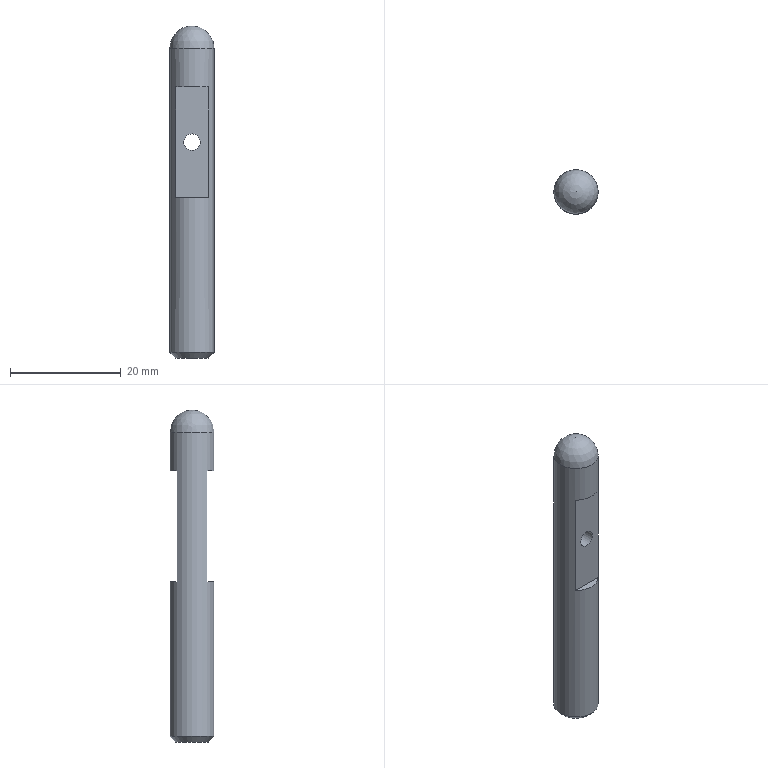Component | NX | ADJ_SUPPORT | 1 solid | 11 faces | box 8 x 8 x 60 mm | volume 2687 mm3 | plane 7 | cylinder 2 | sphere 1 | cone 1 | commonest cylinder face diameters 8 x1 3 x1
STEP:
#1=CARTESIAN_POINT('',(0.,0.,0.));
#2=DIRECTION('',(0.,0.,1.));
#3=DIRECTION('',(1.,0.,0.));
#4=AXIS2_PLACEMENT_3D('',#1,#2,#3);
#5=CARTESIAN_POINT('',(-84.,70.,-253.));
#6=VERTEX_POINT('',#5);
#7=CARTESIAN_POINT('',(-92.,70.,-253.));
#8=VERTEX_POINT('',#7);
#9=CARTESIAN_POINT('',(-88.,70.,-253.));
#10=DIRECTION('',(0.,0.,1.));
#11=DIRECTION('',(1.,0.,0.));
#12=AXIS2_PLACEMENT_3D('',#9,#10,#11);
#13=CIRCLE('',#12,4.);
#14=CARTESIAN_POINT('',(-88.,70.,-254.));
#15=DIRECTION('',(0.,0.,1.));
#16=DIRECTION('',(-1.,0.,0.));
#17=AXIS2_PLACEMENT_3D('',#14,#15,#16);
#18=CYLINDRICAL_SURFACE('',#17,4.);
#19=CARTESIAN_POINT('',(3.142,1.));
#20=DIRECTION('',(1.,0.));
#21=VECTOR('',#20,1.);
#22=LINE('',#19,#21);
#23=(GEOMETRIC_REPRESENTATION_CONTEXT(2)PARAMETRIC_REPRESENTATION_CONTEXT()REPRESENTATION_CONTEXT('',''));
#24=DEFINITIONAL_REPRESENTATION('',(#22),#23);
#25=PCURVE('',#18,#24);
#26=CARTESIAN_POINT('',(-88.,70.,-253.));
#27=DIRECTION('',(0.,0.,1.));
#28=DIRECTION('',(-1.,0.,0.));
#29=AXIS2_PLACEMENT_3D('',#26,#27,#28);
#30=CONICAL_SURFACE('',#29,4.,0.7854);
#31=CARTESIAN_POINT('',(3.142,0.));
#32=DIRECTION('',(1.,0.));
#33=VECTOR('',#32,1.);
#34=LINE('',#31,#33);
#35=(GEOMETRIC_REPRESENTATION_CONTEXT(2)PARAMETRIC_REPRESENTATION_CONTEXT()REPRESENTATION_CONTEXT('',''));
#36=DEFINITIONAL_REPRESENTATION('',(#34),#35);
#37=PCURVE('',#30,#36);
#38=SURFACE_CURVE('',#13,(#25,#37),.PCURVE_S1.);
#39=EDGE_CURVE('',#6,#8,#38,.T.);
#40=ORIENTED_EDGE('',*,*,#39,.T.);
#41=CARTESIAN_POINT('',(-92.,70.,-198.));
#42=VERTEX_POINT('',#41);
#43=CARTESIAN_POINT('',(-92.,70.,-253.));
#44=CARTESIAN_POINT('',(-92.,70.,-198.));
#45=B_SPLINE_CURVE_WITH_KNOTS('',1,(#43,#44),.UNSPECIFIED.,.F.,.F.,(2,2),(1.,56.),.PIECEWISE_BEZIER_KNOTS.);
#46=CARTESIAN_POINT('',(6.283,0.));
#47=DIRECTION('',(0.,1.));
#48=VECTOR('',#47,1.);
#49=LINE('',#46,#48);
#50=(GEOMETRIC_REPRESENTATION_CONTEXT(2)PARAMETRIC_REPRESENTATION_CONTEXT()REPRESENTATION_CONTEXT('',''));
#51=DEFINITIONAL_REPRESENTATION('',(#49),#50);
#52=PCURVE('',#18,#51);
#53=CARTESIAN_POINT('',(0.,0.));
#54=DIRECTION('',(0.,1.));
#55=VECTOR('',#54,1.);
#56=LINE('',#53,#55);
#57=(GEOMETRIC_REPRESENTATION_CONTEXT(2)PARAMETRIC_REPRESENTATION_CONTEXT()REPRESENTATION_CONTEXT('',''));
#58=DEFINITIONAL_REPRESENTATION('',(#56),#57);
#59=PCURVE('',#18,#58);
#60=SEAM_CURVE('',#45,(#52,#59),.PCURVE_S1.);
#61=EDGE_CURVE('',#8,#42,#60,.T.);
#62=ORIENTED_EDGE('',*,*,#61,.T.);
#63=CARTESIAN_POINT('',(-88.,70.,-198.));
#64=DIRECTION('',(0.,0.,-1.));
#65=DIRECTION('',(-1.,0.,0.));
#66=AXIS2_PLACEMENT_3D('',#63,#64,#65);
#67=CIRCLE('',#66,4.);
#68=CARTESIAN_POINT('',(6.283,56.));
#69=DIRECTION('',(-1.,0.));
#70=VECTOR('',#69,1.);
#71=LINE('',#68,#70);
#72=(GEOMETRIC_REPRESENTATION_CONTEXT(2)PARAMETRIC_REPRESENTATION_CONTEXT()REPRESENTATION_CONTEXT('',''));
#73=DEFINITIONAL_REPRESENTATION('',(#71),#72);
#74=PCURVE('',#18,#73);
#75=CARTESIAN_POINT('',(-88.,70.,-198.));
#76=DIRECTION('',(0.,0.,1.));
#77=DIRECTION('',(-1.,0.,0.));
#78=AXIS2_PLACEMENT_3D('',#75,#76,#77);
#79=SPHERICAL_SURFACE('',#78,4.);
#80=CARTESIAN_POINT('',(6.283,0.));
#81=CARTESIAN_POINT('',(6.188,0.));
#82=CARTESIAN_POINT('',(5.998,0.));
#83=CARTESIAN_POINT('',(5.712,0.));
#84=CARTESIAN_POINT('',(5.426,0.));
#85=CARTESIAN_POINT('',(5.141,0.));
#86=CARTESIAN_POINT('',(4.855,0.));
#87=CARTESIAN_POINT('',(4.57,0.));
#88=CARTESIAN_POINT('',(4.284,0.));
#89=CARTESIAN_POINT('',(3.998,0.));
#90=CARTESIAN_POINT('',(3.713,0.));
#91=CARTESIAN_POINT('',(3.427,0.));
#92=CARTESIAN_POINT('',(3.142,0.));
#93=CARTESIAN_POINT('',(2.856,0.));
#94=CARTESIAN_POINT('',(2.57,0.));
#95=CARTESIAN_POINT('',(2.285,0.));
#96=CARTESIAN_POINT('',(1.999,0.));
#97=CARTESIAN_POINT('',(1.714,0.));
#98=CARTESIAN_POINT('',(1.428,0.));
#99=CARTESIAN_POINT('',(1.142,0.));
#100=CARTESIAN_POINT('',(0.8568,0.));
#101=CARTESIAN_POINT('',(0.5712,0.));
#102=CARTESIAN_POINT('',(0.2856,0.));
#103=CARTESIAN_POINT('',(0.0952,0.));
#104=CARTESIAN_POINT('',(0.,0.));
#105=B_SPLINE_CURVE_WITH_KNOTS('',3,(#80,#81,#82,#83,#84,#85,#86,#87,#88,#89,#90,#91,#92,#93,#94,#95,#96,#97,#98,#99,#100,#101,#102,#103,#104),.UNSPECIFIED.,.F.,.F.,(4,1,1,1,1,1,1,1,1,1,1,1,1,1,1,1,1,1,1,1,1,1,4),(0.,0.2856,0.5712,0.8568,1.142,1.428,1.714,1.999,2.285,2.57,2.856,3.142,3.427,3.713,3.998,4.284,4.57,4.855,5.141,5.426,5.712,5.998,6.283),.QUASI_UNIFORM_KNOTS.);
#106=(GEOMETRIC_REPRESENTATION_CONTEXT(2)PARAMETRIC_REPRESENTATION_CONTEXT()REPRESENTATION_CONTEXT('',''));
#107=DEFINITIONAL_REPRESENTATION('',(#105),#106);
#108=PCURVE('',#79,#107);
#109=SURFACE_CURVE('',#67,(#74,#108),.PCURVE_S1.);
#110=EDGE_CURVE('',#42,#42,#109,.T.);
#111=ORIENTED_EDGE('',*,*,#110,.T.);
#112=ORIENTED_EDGE('',*,*,#61,.F.);
#113=CARTESIAN_POINT('',(-88.,70.,-253.));
#114=DIRECTION('',(0.,0.,1.));
#115=DIRECTION('',(1.,0.,0.));
#116=AXIS2_PLACEMENT_3D('',#113,#114,#115);
#117=CIRCLE('',#116,4.);
#118=CARTESIAN_POINT('',(-3.142,1.));
#119=DIRECTION('',(1.,0.));
#120=VECTOR('',#119,1.);
#121=LINE('',#118,#120);
#122=(GEOMETRIC_REPRESENTATION_CONTEXT(2)PARAMETRIC_REPRESENTATION_CONTEXT()REPRESENTATION_CONTEXT('',''));
#123=DEFINITIONAL_REPRESENTATION('',(#121),#122);
#124=PCURVE('',#18,#123);
#125=CARTESIAN_POINT('',(3.142,0.));
#126=DIRECTION('',(1.,0.));
#127=VECTOR('',#126,1.);
#128=LINE('',#125,#127);
#129=(GEOMETRIC_REPRESENTATION_CONTEXT(2)PARAMETRIC_REPRESENTATION_CONTEXT()REPRESENTATION_CONTEXT('',''));
#130=DEFINITIONAL_REPRESENTATION('',(#128),#129);
#131=PCURVE('',#30,#130);
#132=SURFACE_CURVE('',#117,(#124,#131),.PCURVE_S1.);
#133=EDGE_CURVE('',#8,#6,#132,.T.);
#134=ORIENTED_EDGE('',*,*,#133,.T.);
#135=EDGE_LOOP('',(#40,#62,#111,#112,#134));
#136=FACE_BOUND('',#135,.T.);
#137=CARTESIAN_POINT('',(-85.049,67.3,-205.));
#138=VERTEX_POINT('',#137);
#139=CARTESIAN_POINT('',(-85.049,67.3,-225.));
#140=VERTEX_POINT('',#139);
#141=CARTESIAN_POINT('',(-85.049,67.3,-254.));
#142=DIRECTION('',(0.,0.,-1.));
#143=VECTOR('',#142,1.);
#144=LINE('',#141,#143);
#145=CARTESIAN_POINT('',(2.401,0.));
#146=DIRECTION('',(0.,-1.));
#147=VECTOR('',#146,1.);
#148=LINE('',#145,#147);
#149=(GEOMETRIC_REPRESENTATION_CONTEXT(2)PARAMETRIC_REPRESENTATION_CONTEXT()REPRESENTATION_CONTEXT('',''));
#150=DEFINITIONAL_REPRESENTATION('',(#148),#149);
#151=PCURVE('',#18,#150);
#152=CARTESIAN_POINT('',(-108.,67.3,-205.));
#153=DIRECTION('',(0.,-1.,0.));
#154=DIRECTION('',(0.,0.,1.));
#155=AXIS2_PLACEMENT_3D('',#152,#153,#154);
#156=PLANE('',#155);
#157=CARTESIAN_POINT('',(-49.,-22.951));
#158=DIRECTION('',(-1.,0.));
#159=VECTOR('',#158,1.);
#160=LINE('',#157,#159);
#161=(GEOMETRIC_REPRESENTATION_CONTEXT(2)PARAMETRIC_REPRESENTATION_CONTEXT()REPRESENTATION_CONTEXT('',''));
#162=DEFINITIONAL_REPRESENTATION('',(#160),#161);
#163=PCURVE('',#156,#162);
#164=SURFACE_CURVE('',#144,(#151,#163),.PCURVE_S1.);
#165=EDGE_CURVE('',#138,#140,#164,.T.);
#166=ORIENTED_EDGE('',*,*,#165,.T.);
#167=CARTESIAN_POINT('',(-90.951,67.3,-225.));
#168=VERTEX_POINT('',#167);
#169=CARTESIAN_POINT('',(-88.,70.,-225.));
#170=DIRECTION('',(0.,0.,-1.));
#171=DIRECTION('',(-1.,0.,0.));
#172=AXIS2_PLACEMENT_3D('',#169,#170,#171);
#173=CIRCLE('',#172,4.);
#174=CARTESIAN_POINT('',(6.283,29.));
#175=DIRECTION('',(-1.,0.));
#176=VECTOR('',#175,1.);
#177=LINE('',#174,#176);
#178=(GEOMETRIC_REPRESENTATION_CONTEXT(2)PARAMETRIC_REPRESENTATION_CONTEXT()REPRESENTATION_CONTEXT('',''));
#179=DEFINITIONAL_REPRESENTATION('',(#177),#178);
#180=PCURVE('',#18,#179);
#181=CARTESIAN_POINT('',(-108.,67.3,-225.));
#182=DIRECTION('',(0.,0.,1.));
#183=DIRECTION('',(-1.,0.,0.));
#184=AXIS2_PLACEMENT_3D('',#181,#182,#183);
#185=PLANE('',#184);
#186=CARTESIAN_POINT('',(-16.,-2.7));
#187=CARTESIAN_POINT('',(-16.,-9.628));
#188=CARTESIAN_POINT('',(-22.,-6.164));
#189=CARTESIAN_POINT('',(-28.,-2.7));
#190=CARTESIAN_POINT('',(-22.,0.7641));
#191=CARTESIAN_POINT('',(-16.,4.228));
#192=CARTESIAN_POINT('',(-16.,-2.7));
#193=(BOUNDED_CURVE()B_SPLINE_CURVE(2,(#186,#187,#188,#189,#190,#191,#192),.UNSPECIFIED.,.T.,.F.)B_SPLINE_CURVE_WITH_KNOTS((1,2,2,2,2,1),(-2.094,0.,2.094,4.189,6.283,8.378),.UNSPECIFIED.)CURVE()GEOMETRIC_REPRESENTATION_ITEM()RATIONAL_B_SPLINE_CURVE((1.,0.5,1.,0.5,1.,0.5,1.))REPRESENTATION_ITEM(''));
#194=(GEOMETRIC_REPRESENTATION_CONTEXT(2)PARAMETRIC_REPRESENTATION_CONTEXT()REPRESENTATION_CONTEXT('',''));
#195=DEFINITIONAL_REPRESENTATION('',(#193),#194);
#196=PCURVE('',#185,#195);
#197=SURFACE_CURVE('',#173,(#180,#196),.PCURVE_S1.);
#198=EDGE_CURVE('',#140,#168,#197,.T.);
#199=ORIENTED_EDGE('',*,*,#198,.T.);
#200=CARTESIAN_POINT('',(-90.951,67.3,-205.));
#201=VERTEX_POINT('',#200);
#202=CARTESIAN_POINT('',(-90.951,67.3,-254.));
#203=DIRECTION('',(0.,0.,1.));
#204=VECTOR('',#203,1.);
#205=LINE('',#202,#204);
#206=CARTESIAN_POINT('',(0.741,0.));
#207=DIRECTION('',(0.,1.));
#208=VECTOR('',#207,1.);
#209=LINE('',#206,#208);
#210=(GEOMETRIC_REPRESENTATION_CONTEXT(2)PARAMETRIC_REPRESENTATION_CONTEXT()REPRESENTATION_CONTEXT('',''));
#211=DEFINITIONAL_REPRESENTATION('',(#209),#210);
#212=PCURVE('',#18,#211);
#213=CARTESIAN_POINT('',(-49.,-17.049));
#214=DIRECTION('',(1.,0.));
#215=VECTOR('',#214,1.);
#216=LINE('',#213,#215);
#217=(GEOMETRIC_REPRESENTATION_CONTEXT(2)PARAMETRIC_REPRESENTATION_CONTEXT()REPRESENTATION_CONTEXT('',''));
#218=DEFINITIONAL_REPRESENTATION('',(#216),#217);
#219=PCURVE('',#156,#218);
#220=SURFACE_CURVE('',#205,(#212,#219),.PCURVE_S1.);
#221=EDGE_CURVE('',#168,#201,#220,.T.);
#222=ORIENTED_EDGE('',*,*,#221,.T.);
#223=CARTESIAN_POINT('',(-88.,70.,-205.));
#224=DIRECTION('',(0.,0.,1.));
#225=DIRECTION('',(1.,0.,0.));
#226=AXIS2_PLACEMENT_3D('',#223,#224,#225);
#227=CIRCLE('',#226,4.);
#228=CARTESIAN_POINT('',(-3.142,49.));
#229=DIRECTION('',(1.,0.));
#230=VECTOR('',#229,1.);
#231=LINE('',#228,#230);
#232=(GEOMETRIC_REPRESENTATION_CONTEXT(2)PARAMETRIC_REPRESENTATION_CONTEXT()REPRESENTATION_CONTEXT('',''));
#233=DEFINITIONAL_REPRESENTATION('',(#231),#232);
#234=PCURVE('',#18,#233);
#235=CARTESIAN_POINT('',(-108.,60.,-205.));
#236=DIRECTION('',(0.,0.,-1.));
#237=DIRECTION('',(1.,0.,0.));
#238=AXIS2_PLACEMENT_3D('',#235,#236,#237);
#239=PLANE('',#238);
#240=CARTESIAN_POINT('',(24.,-10.));
#241=CARTESIAN_POINT('',(24.,-16.928));
#242=CARTESIAN_POINT('',(18.,-13.464));
#243=CARTESIAN_POINT('',(12.,-10.));
#244=CARTESIAN_POINT('',(18.,-6.536));
#245=CARTESIAN_POINT('',(24.,-3.072));
#246=CARTESIAN_POINT('',(24.,-10.));
#247=(BOUNDED_CURVE()B_SPLINE_CURVE(2,(#240,#241,#242,#243,#244,#245,#246),.UNSPECIFIED.,.T.,.F.)B_SPLINE_CURVE_WITH_KNOTS((1,2,2,2,2,1),(-2.094,0.,2.094,4.189,6.283,8.378),.UNSPECIFIED.)CURVE()GEOMETRIC_REPRESENTATION_ITEM()RATIONAL_B_SPLINE_CURVE((1.,0.5,1.,0.5,1.,0.5,1.))REPRESENTATION_ITEM(''));
#248=(GEOMETRIC_REPRESENTATION_CONTEXT(2)PARAMETRIC_REPRESENTATION_CONTEXT()REPRESENTATION_CONTEXT('',''));
#249=DEFINITIONAL_REPRESENTATION('',(#247),#248);
#250=PCURVE('',#239,#249);
#251=SURFACE_CURVE('',#227,(#234,#250),.PCURVE_S1.);
#252=EDGE_CURVE('',#201,#138,#251,.T.);
#253=ORIENTED_EDGE('',*,*,#252,.T.);
#254=EDGE_LOOP('',(#166,#199,#222,#253));
#255=FACE_BOUND('',#254,.T.);
#256=CARTESIAN_POINT('',(-90.951,72.7,-205.));
#257=VERTEX_POINT('',#256);
#258=CARTESIAN_POINT('',(-90.951,72.7,-225.));
#259=VERTEX_POINT('',#258);
#260=CARTESIAN_POINT('',(-90.951,72.7,-254.));
#261=DIRECTION('',(0.,0.,-1.));
#262=VECTOR('',#261,1.);
#263=LINE('',#260,#262);
#264=CARTESIAN_POINT('',(5.542,0.));
#265=DIRECTION('',(0.,-1.));
#266=VECTOR('',#265,1.);
#267=LINE('',#264,#266);
#268=(GEOMETRIC_REPRESENTATION_CONTEXT(2)PARAMETRIC_REPRESENTATION_CONTEXT()REPRESENTATION_CONTEXT('',''));
#269=DEFINITIONAL_REPRESENTATION('',(#267),#268);
#270=PCURVE('',#18,#269);
#271=CARTESIAN_POINT('',(-108.,72.7,-225.));
#272=DIRECTION('',(0.,1.,0.));
#273=DIRECTION('',(0.,0.,-1.));
#274=AXIS2_PLACEMENT_3D('',#271,#272,#273);
#275=PLANE('',#274);
#276=CARTESIAN_POINT('',(29.,-17.049));
#277=DIRECTION('',(1.,0.));
#278=VECTOR('',#277,1.);
#279=LINE('',#276,#278);
#280=(GEOMETRIC_REPRESENTATION_CONTEXT(2)PARAMETRIC_REPRESENTATION_CONTEXT()REPRESENTATION_CONTEXT('',''));
#281=DEFINITIONAL_REPRESENTATION('',(#279),#280);
#282=PCURVE('',#275,#281);
#283=SURFACE_CURVE('',#263,(#270,#282),.PCURVE_S1.);
#284=EDGE_CURVE('',#257,#259,#283,.T.);
#285=ORIENTED_EDGE('',*,*,#284,.T.);
#286=CARTESIAN_POINT('',(-85.049,72.7,-225.));
#287=VERTEX_POINT('',#286);
#288=CARTESIAN_POINT('',(-88.,70.,-225.));
#289=DIRECTION('',(0.,0.,-1.));
#290=DIRECTION('',(-1.,0.,0.));
#291=AXIS2_PLACEMENT_3D('',#288,#289,#290);
#292=CIRCLE('',#291,4.);
#293=CARTESIAN_POINT('',(6.283,29.));
#294=DIRECTION('',(-1.,0.));
#295=VECTOR('',#294,1.);
#296=LINE('',#293,#295);
#297=(GEOMETRIC_REPRESENTATION_CONTEXT(2)PARAMETRIC_REPRESENTATION_CONTEXT()REPRESENTATION_CONTEXT('',''));
#298=DEFINITIONAL_REPRESENTATION('',(#296),#297);
#299=PCURVE('',#18,#298);
#300=CARTESIAN_POINT('',(-108.,80.,-225.));
#301=DIRECTION('',(0.,0.,1.));
#302=DIRECTION('',(-1.,0.,0.));
#303=AXIS2_PLACEMENT_3D('',#300,#301,#302);
#304=PLANE('',#303);
#305=CARTESIAN_POINT('',(-16.,10.));
#306=CARTESIAN_POINT('',(-16.,3.072));
#307=CARTESIAN_POINT('',(-22.,6.536));
#308=CARTESIAN_POINT('',(-28.,10.));
#309=CARTESIAN_POINT('',(-22.,13.464));
#310=CARTESIAN_POINT('',(-16.,16.928));
#311=CARTESIAN_POINT('',(-16.,10.));
#312=(BOUNDED_CURVE()B_SPLINE_CURVE(2,(#305,#306,#307,#308,#309,#310,#311),.UNSPECIFIED.,.T.,.F.)B_SPLINE_CURVE_WITH_KNOTS((1,2,2,2,2,1),(-2.094,0.,2.094,4.189,6.283,8.378),.UNSPECIFIED.)CURVE()GEOMETRIC_REPRESENTATION_ITEM()RATIONAL_B_SPLINE_CURVE((1.,0.5,1.,0.5,1.,0.5,1.))REPRESENTATION_ITEM(''));
#313=(GEOMETRIC_REPRESENTATION_CONTEXT(2)PARAMETRIC_REPRESENTATION_CONTEXT()REPRESENTATION_CONTEXT('',''));
#314=DEFINITIONAL_REPRESENTATION('',(#312),#313);
#315=PCURVE('',#304,#314);
#316=SURFACE_CURVE('',#292,(#299,#315),.PCURVE_S1.);
#317=EDGE_CURVE('',#259,#287,#316,.T.);
#318=ORIENTED_EDGE('',*,*,#317,.T.);
#319=CARTESIAN_POINT('',(-85.049,72.7,-205.));
#320=VERTEX_POINT('',#319);
#321=CARTESIAN_POINT('',(-85.049,72.7,-254.));
#322=DIRECTION('',(0.,0.,1.));
#323=VECTOR('',#322,1.);
#324=LINE('',#321,#323);
#325=CARTESIAN_POINT('',(3.883,0.));
#326=DIRECTION('',(0.,1.));
#327=VECTOR('',#326,1.);
#328=LINE('',#325,#327);
#329=(GEOMETRIC_REPRESENTATION_CONTEXT(2)PARAMETRIC_REPRESENTATION_CONTEXT()REPRESENTATION_CONTEXT('',''));
#330=DEFINITIONAL_REPRESENTATION('',(#328),#329);
#331=PCURVE('',#18,#330);
#332=CARTESIAN_POINT('',(29.,-22.951));
#333=DIRECTION('',(-1.,0.));
#334=VECTOR('',#333,1.);
#335=LINE('',#332,#334);
#336=(GEOMETRIC_REPRESENTATION_CONTEXT(2)PARAMETRIC_REPRESENTATION_CONTEXT()REPRESENTATION_CONTEXT('',''));
#337=DEFINITIONAL_REPRESENTATION('',(#335),#336);
#338=PCURVE('',#275,#337);
#339=SURFACE_CURVE('',#324,(#331,#338),.PCURVE_S1.);
#340=EDGE_CURVE('',#287,#320,#339,.T.);
#341=ORIENTED_EDGE('',*,*,#340,.T.);
#342=CARTESIAN_POINT('',(-88.,70.,-205.));
#343=DIRECTION('',(0.,0.,1.));
#344=DIRECTION('',(1.,0.,0.));
#345=AXIS2_PLACEMENT_3D('',#342,#343,#344);
#346=CIRCLE('',#345,4.);
#347=CARTESIAN_POINT('',(3.142,49.));
#348=DIRECTION('',(1.,0.));
#349=VECTOR('',#348,1.);
#350=LINE('',#347,#349);
#351=(GEOMETRIC_REPRESENTATION_CONTEXT(2)PARAMETRIC_REPRESENTATION_CONTEXT()REPRESENTATION_CONTEXT('',''));
#352=DEFINITIONAL_REPRESENTATION('',(#350),#351);
#353=PCURVE('',#18,#352);
#354=CARTESIAN_POINT('',(-108.,72.7,-205.));
#355=DIRECTION('',(0.,0.,-1.));
#356=DIRECTION('',(1.,0.,0.));
#357=AXIS2_PLACEMENT_3D('',#354,#355,#356);
#358=PLANE('',#357);
#359=CARTESIAN_POINT('',(24.,2.7));
#360=CARTESIAN_POINT('',(24.,-4.228));
#361=CARTESIAN_POINT('',(18.,-0.7641));
#362=CARTESIAN_POINT('',(12.,2.7));
#363=CARTESIAN_POINT('',(18.,6.164));
#364=CARTESIAN_POINT('',(24.,9.628));
#365=CARTESIAN_POINT('',(24.,2.7));
#366=(BOUNDED_CURVE()B_SPLINE_CURVE(2,(#359,#360,#361,#362,#363,#364,#365),.UNSPECIFIED.,.T.,.F.)B_SPLINE_CURVE_WITH_KNOTS((1,2,2,2,2,1),(-2.094,0.,2.094,4.189,6.283,8.378),.UNSPECIFIED.)CURVE()GEOMETRIC_REPRESENTATION_ITEM()RATIONAL_B_SPLINE_CURVE((1.,0.5,1.,0.5,1.,0.5,1.))REPRESENTATION_ITEM(''));
#367=(GEOMETRIC_REPRESENTATION_CONTEXT(2)PARAMETRIC_REPRESENTATION_CONTEXT()REPRESENTATION_CONTEXT('',''));
#368=DEFINITIONAL_REPRESENTATION('',(#366),#367);
#369=PCURVE('',#358,#368);
#370=SURFACE_CURVE('',#346,(#353,#369),.PCURVE_S1.);
#371=EDGE_CURVE('',#320,#257,#370,.T.);
#372=ORIENTED_EDGE('',*,*,#371,.T.);
#373=EDGE_LOOP('',(#285,#318,#341,#372));
#374=FACE_BOUND('',#373,.T.);
#375=ADVANCED_FACE('',(#136,#255,#374),#18,.T.);
#376=CARTESIAN_POINT('',(-85.,70.,-254.));
#377=VERTEX_POINT('',#376);
#378=CARTESIAN_POINT('',(-88.,70.,-254.));
#379=DIRECTION('',(0.,0.,-1.));
#380=DIRECTION('',(1.,0.,0.));
#381=AXIS2_PLACEMENT_3D('',#378,#379,#380);
#382=CIRCLE('',#381,3.);
#383=CARTESIAN_POINT('',(-88.,70.,-254.));
#384=DIRECTION('',(0.,0.,-1.));
#385=DIRECTION('',(1.,0.,0.));
#386=AXIS2_PLACEMENT_3D('',#383,#384,#385);
#387=PLANE('',#386);
#388=CARTESIAN_POINT('',(0.,0.));
#389=DIRECTION('',(1.,0.));
#390=AXIS2_PLACEMENT_2D('',#388,#389);
#391=CIRCLE('',#390,3.);
#392=(GEOMETRIC_REPRESENTATION_CONTEXT(2)PARAMETRIC_REPRESENTATION_CONTEXT()REPRESENTATION_CONTEXT('',''));
#393=DEFINITIONAL_REPRESENTATION('',(#391),#392);
#394=PCURVE('',#387,#393);
#395=CARTESIAN_POINT('',(9.425,-1.));
#396=DIRECTION('',(-1.,0.));
#397=VECTOR('',#396,1.);
#398=LINE('',#395,#397);
#399=(GEOMETRIC_REPRESENTATION_CONTEXT(2)PARAMETRIC_REPRESENTATION_CONTEXT()REPRESENTATION_CONTEXT('',''));
#400=DEFINITIONAL_REPRESENTATION('',(#398),#399);
#401=PCURVE('',#30,#400);
#402=SURFACE_CURVE('',#382,(#394,#401),.PCURVE_S1.);
#403=EDGE_CURVE('',#377,#377,#402,.T.);
#404=ORIENTED_EDGE('',*,*,#403,.T.);
#405=EDGE_LOOP('',(#404));
#406=FACE_BOUND('',#405,.T.);
#407=ADVANCED_FACE('',(#406),#387,.T.);
#408=ORIENTED_EDGE('',*,*,#110,.F.);
#409=CARTESIAN_POINT('',(-88.,70.,-194.));
#410=VERTEX_POINT('',#409);
#411=CARTESIAN_POINT('',(-92.,70.,-198.));
#412=CARTESIAN_POINT('',(-92.,70.,-196.953));
#413=CARTESIAN_POINT('',(-91.671,70.,-195.906));
#414=CARTESIAN_POINT('',(-91.013,70.,-194.987));
#415=CARTESIAN_POINT('',(-90.094,70.,-194.329));
#416=CARTESIAN_POINT('',(-89.047,70.,-194.));
#417=CARTESIAN_POINT('',(-88.,70.,-194.));
#418=B_SPLINE_CURVE_WITH_KNOTS('',6,(#411,#412,#413,#414,#415,#416,#417),.UNSPECIFIED.,.F.,.F.,(7,7),(0.,1.571),.PIECEWISE_BEZIER_KNOTS.);
#419=CARTESIAN_POINT('',(6.283,0.));
#420=DIRECTION('',(0.,1.));
#421=VECTOR('',#420,1.);
#422=LINE('',#419,#421);
#423=(GEOMETRIC_REPRESENTATION_CONTEXT(2)PARAMETRIC_REPRESENTATION_CONTEXT()REPRESENTATION_CONTEXT('',''));
#424=DEFINITIONAL_REPRESENTATION('',(#422),#423);
#425=PCURVE('',#79,#424);
#426=CARTESIAN_POINT('',(0.,0.));
#427=DIRECTION('',(0.,1.));
#428=VECTOR('',#427,1.);
#429=LINE('',#426,#428);
#430=(GEOMETRIC_REPRESENTATION_CONTEXT(2)PARAMETRIC_REPRESENTATION_CONTEXT()REPRESENTATION_CONTEXT('',''));
#431=DEFINITIONAL_REPRESENTATION('',(#429),#430);
#432=PCURVE('',#79,#431);
#433=SEAM_CURVE('',#418,(#425,#432),.PCURVE_S1.);
#434=EDGE_CURVE('',#42,#410,#433,.T.);
#435=ORIENTED_EDGE('',*,*,#434,.T.);
#436=ORIENTED_EDGE('',*,*,#434,.F.);
#437=EDGE_LOOP('',(#408,#435,#436));
#438=FACE_BOUND('',#437,.T.);
#439=ADVANCED_FACE('',(#438),#79,.T.);
#440=CARTESIAN_POINT('',(-88.,67.3,-213.5));
#441=VERTEX_POINT('',#440);
#442=CARTESIAN_POINT('',(-88.,67.3,-215.));
#443=DIRECTION('',(0.,-1.,0.));
#444=DIRECTION('',(0.,0.,1.));
#445=AXIS2_PLACEMENT_3D('',#442,#443,#444);
#446=CIRCLE('',#445,1.5);
#447=CARTESIAN_POINT('',(-10.,-20.));
#448=DIRECTION('',(1.,0.));
#449=AXIS2_PLACEMENT_2D('',#447,#448);
#450=CIRCLE('',#449,1.5);
#451=(GEOMETRIC_REPRESENTATION_CONTEXT(2)PARAMETRIC_REPRESENTATION_CONTEXT()REPRESENTATION_CONTEXT('',''));
#452=DEFINITIONAL_REPRESENTATION('',(#450),#451);
#453=PCURVE('',#156,#452);
#454=CARTESIAN_POINT('',(-88.,72.7,-215.));
#455=DIRECTION('',(0.,-1.,-0.));
#456=DIRECTION('',(0.,-0.,1.));
#457=AXIS2_PLACEMENT_3D('',#454,#455,#456);
#458=CYLINDRICAL_SURFACE('',#457,1.5);
#459=CARTESIAN_POINT('',(0.,5.4));
#460=DIRECTION('',(1.,0.));
#461=VECTOR('',#460,1.);
#462=LINE('',#459,#461);
#463=(GEOMETRIC_REPRESENTATION_CONTEXT(2)PARAMETRIC_REPRESENTATION_CONTEXT()REPRESENTATION_CONTEXT('',''));
#464=DEFINITIONAL_REPRESENTATION('',(#462),#463);
#465=PCURVE('',#458,#464);
#466=SURFACE_CURVE('',#446,(#453,#465),.PCURVE_S1.);
#467=EDGE_CURVE('',#441,#441,#466,.T.);
#468=ORIENTED_EDGE('',*,*,#467,.F.);
#469=EDGE_LOOP('',(#468));
#470=FACE_BOUND('',#469,.T.);
#471=CARTESIAN_POINT('',(-108.,67.3,-205.));
#472=DIRECTION('',(-1.,0.,0.));
#473=VECTOR('',#472,1.);
#474=LINE('',#471,#473);
#475=CARTESIAN_POINT('',(0.,0.));
#476=DIRECTION('',(0.,1.));
#477=VECTOR('',#476,1.);
#478=LINE('',#475,#477);
#479=(GEOMETRIC_REPRESENTATION_CONTEXT(2)PARAMETRIC_REPRESENTATION_CONTEXT()REPRESENTATION_CONTEXT('',''));
#480=DEFINITIONAL_REPRESENTATION('',(#478),#479);
#481=PCURVE('',#156,#480);
#482=CARTESIAN_POINT('',(0.,-7.3));
#483=DIRECTION('',(-1.,0.));
#484=VECTOR('',#483,1.);
#485=LINE('',#482,#484);
#486=(GEOMETRIC_REPRESENTATION_CONTEXT(2)PARAMETRIC_REPRESENTATION_CONTEXT()REPRESENTATION_CONTEXT('',''));
#487=DEFINITIONAL_REPRESENTATION('',(#485),#486);
#488=PCURVE('',#239,#487);
#489=SURFACE_CURVE('',#474,(#481,#488),.PCURVE_S1.);
#490=EDGE_CURVE('',#138,#201,#489,.T.);
#491=ORIENTED_EDGE('',*,*,#490,.T.);
#492=ORIENTED_EDGE('',*,*,#221,.F.);
#493=CARTESIAN_POINT('',(-108.,67.3,-225.));
#494=DIRECTION('',(-1.,0.,0.));
#495=VECTOR('',#494,1.);
#496=LINE('',#493,#495);
#497=CARTESIAN_POINT('',(-20.,0.));
#498=DIRECTION('',(0.,1.));
#499=VECTOR('',#498,1.);
#500=LINE('',#497,#499);
#501=(GEOMETRIC_REPRESENTATION_CONTEXT(2)PARAMETRIC_REPRESENTATION_CONTEXT()REPRESENTATION_CONTEXT('',''));
#502=DEFINITIONAL_REPRESENTATION('',(#500),#501);
#503=PCURVE('',#156,#502);
#504=CARTESIAN_POINT('',(0.,0.));
#505=DIRECTION('',(1.,0.));
#506=VECTOR('',#505,1.);
#507=LINE('',#504,#506);
#508=(GEOMETRIC_REPRESENTATION_CONTEXT(2)PARAMETRIC_REPRESENTATION_CONTEXT()REPRESENTATION_CONTEXT('',''));
#509=DEFINITIONAL_REPRESENTATION('',(#507),#508);
#510=PCURVE('',#185,#509);
#511=SURFACE_CURVE('',#496,(#503,#510),.PCURVE_S1.);
#512=EDGE_CURVE('',#140,#168,#511,.T.);
#513=ORIENTED_EDGE('',*,*,#512,.F.);
#514=ORIENTED_EDGE('',*,*,#165,.F.);
#515=EDGE_LOOP('',(#491,#492,#513,#514));
#516=FACE_BOUND('',#515,.T.);
#517=ADVANCED_FACE('',(#470,#516),#156,.T.);
#518=ORIENTED_EDGE('',*,*,#512,.T.);
#519=ORIENTED_EDGE('',*,*,#198,.F.);
#520=EDGE_LOOP('',(#518,#519));
#521=FACE_BOUND('',#520,.T.);
#522=ADVANCED_FACE('',(#521),#185,.T.);
#523=ORIENTED_EDGE('',*,*,#490,.F.);
#524=ORIENTED_EDGE('',*,*,#252,.F.);
#525=EDGE_LOOP('',(#523,#524));
#526=FACE_BOUND('',#525,.T.);
#527=ADVANCED_FACE('',(#526),#239,.T.);
#528=CARTESIAN_POINT('',(-108.,72.7,-225.));
#529=DIRECTION('',(-1.,0.,0.));
#530=VECTOR('',#529,1.);
#531=LINE('',#528,#530);
#532=CARTESIAN_POINT('',(0.,7.3));
#533=DIRECTION('',(1.,0.));
#534=VECTOR('',#533,1.);
#535=LINE('',#532,#534);
#536=(GEOMETRIC_REPRESENTATION_CONTEXT(2)PARAMETRIC_REPRESENTATION_CONTEXT()REPRESENTATION_CONTEXT('',''));
#537=DEFINITIONAL_REPRESENTATION('',(#535),#536);
#538=PCURVE('',#304,#537);
#539=CARTESIAN_POINT('',(0.,0.));
#540=DIRECTION('',(0.,1.));
#541=VECTOR('',#540,1.);
#542=LINE('',#539,#541);
#543=(GEOMETRIC_REPRESENTATION_CONTEXT(2)PARAMETRIC_REPRESENTATION_CONTEXT()REPRESENTATION_CONTEXT('',''));
#544=DEFINITIONAL_REPRESENTATION('',(#542),#543);
#545=PCURVE('',#275,#544);
#546=SURFACE_CURVE('',#531,(#538,#545),.PCURVE_S1.);
#547=EDGE_CURVE('',#287,#259,#546,.T.);
#548=ORIENTED_EDGE('',*,*,#547,.F.);
#549=ORIENTED_EDGE('',*,*,#317,.F.);
#550=EDGE_LOOP('',(#548,#549));
#551=FACE_BOUND('',#550,.T.);
#552=ADVANCED_FACE('',(#551),#304,.T.);
#553=CARTESIAN_POINT('',(-88.,72.7,-213.5));
#554=VERTEX_POINT('',#553);
#555=CARTESIAN_POINT('',(-88.,72.7,-215.));
#556=DIRECTION('',(0.,-1.,-0.));
#557=DIRECTION('',(0.,-0.,1.));
#558=AXIS2_PLACEMENT_3D('',#555,#556,#557);
#559=CIRCLE('',#558,1.5);
#560=CARTESIAN_POINT('',(-11.5,-20.));
#561=CARTESIAN_POINT('',(-11.5,-17.402));
#562=CARTESIAN_POINT('',(-9.25,-18.701));
#563=CARTESIAN_POINT('',(-7.,-20.));
#564=CARTESIAN_POINT('',(-9.25,-21.299));
#565=CARTESIAN_POINT('',(-11.5,-22.598));
#566=CARTESIAN_POINT('',(-11.5,-20.));
#567=(BOUNDED_CURVE()B_SPLINE_CURVE(2,(#560,#561,#562,#563,#564,#565,#566),.UNSPECIFIED.,.T.,.F.)B_SPLINE_CURVE_WITH_KNOTS((1,2,2,2,2,1),(-2.094,0.,2.094,4.189,6.283,8.378),.UNSPECIFIED.)CURVE()GEOMETRIC_REPRESENTATION_ITEM()RATIONAL_B_SPLINE_CURVE((1.,0.5,1.,0.5,1.,0.5,1.))REPRESENTATION_ITEM(''));
#568=(GEOMETRIC_REPRESENTATION_CONTEXT(2)PARAMETRIC_REPRESENTATION_CONTEXT()REPRESENTATION_CONTEXT('',''));
#569=DEFINITIONAL_REPRESENTATION('',(#567),#568);
#570=PCURVE('',#275,#569);
#571=CARTESIAN_POINT('',(0.,0.));
#572=DIRECTION('',(1.,0.));
#573=VECTOR('',#572,1.);
#574=LINE('',#571,#573);
#575=(GEOMETRIC_REPRESENTATION_CONTEXT(2)PARAMETRIC_REPRESENTATION_CONTEXT()REPRESENTATION_CONTEXT('',''));
#576=DEFINITIONAL_REPRESENTATION('',(#574),#575);
#577=PCURVE('',#458,#576);
#578=SURFACE_CURVE('',#559,(#570,#577),.PCURVE_S1.);
#579=EDGE_CURVE('',#554,#554,#578,.T.);
#580=ORIENTED_EDGE('',*,*,#579,.T.);
#581=EDGE_LOOP('',(#580));
#582=FACE_BOUND('',#581,.T.);
#583=CARTESIAN_POINT('',(-108.,72.7,-205.));
#584=DIRECTION('',(-1.,0.,0.));
#585=VECTOR('',#584,1.);
#586=LINE('',#583,#585);
#587=CARTESIAN_POINT('',(-20.,0.));
#588=DIRECTION('',(0.,1.));
#589=VECTOR('',#588,1.);
#590=LINE('',#587,#589);
#591=(GEOMETRIC_REPRESENTATION_CONTEXT(2)PARAMETRIC_REPRESENTATION_CONTEXT()REPRESENTATION_CONTEXT('',''));
#592=DEFINITIONAL_REPRESENTATION('',(#590),#591);
#593=PCURVE('',#275,#592);
#594=CARTESIAN_POINT('',(0.,0.));
#595=DIRECTION('',(-1.,0.));
#596=VECTOR('',#595,1.);
#597=LINE('',#594,#596);
#598=(GEOMETRIC_REPRESENTATION_CONTEXT(2)PARAMETRIC_REPRESENTATION_CONTEXT()REPRESENTATION_CONTEXT('',''));
#599=DEFINITIONAL_REPRESENTATION('',(#597),#598);
#600=PCURVE('',#358,#599);
#601=SURFACE_CURVE('',#586,(#593,#600),.PCURVE_S1.);
#602=EDGE_CURVE('',#320,#257,#601,.T.);
#603=ORIENTED_EDGE('',*,*,#602,.F.);
#604=ORIENTED_EDGE('',*,*,#340,.F.);
#605=ORIENTED_EDGE('',*,*,#547,.T.);
#606=ORIENTED_EDGE('',*,*,#284,.F.);
#607=EDGE_LOOP('',(#603,#604,#605,#606));
#608=FACE_BOUND('',#607,.T.);
#609=ADVANCED_FACE('',(#582,#608),#275,.T.);
#610=ORIENTED_EDGE('',*,*,#602,.T.);
#611=ORIENTED_EDGE('',*,*,#371,.F.);
#612=EDGE_LOOP('',(#610,#611));
#613=FACE_BOUND('',#612,.T.);
#614=ADVANCED_FACE('',(#613),#358,.T.);
#615=ORIENTED_EDGE('',*,*,#467,.F.);
#616=CARTESIAN_POINT('',(-88.,72.7,-213.5));
#617=CARTESIAN_POINT('',(-88.,67.3,-213.5));
#618=B_SPLINE_CURVE_WITH_KNOTS('',1,(#616,#617),.UNSPECIFIED.,.F.,.F.,(2,2),(0.,5.4),.PIECEWISE_BEZIER_KNOTS.);
#619=CARTESIAN_POINT('',(0.,0.));
#620=DIRECTION('',(0.,1.));
#621=VECTOR('',#620,1.);
#622=LINE('',#619,#621);
#623=(GEOMETRIC_REPRESENTATION_CONTEXT(2)PARAMETRIC_REPRESENTATION_CONTEXT()REPRESENTATION_CONTEXT('',''));
#624=DEFINITIONAL_REPRESENTATION('',(#622),#623);
#625=PCURVE('',#458,#624);
#626=CARTESIAN_POINT('',(6.283,0.));
#627=DIRECTION('',(0.,1.));
#628=VECTOR('',#627,1.);
#629=LINE('',#626,#628);
#630=(GEOMETRIC_REPRESENTATION_CONTEXT(2)PARAMETRIC_REPRESENTATION_CONTEXT()REPRESENTATION_CONTEXT('',''));
#631=DEFINITIONAL_REPRESENTATION('',(#629),#630);
#632=PCURVE('',#458,#631);
#633=SEAM_CURVE('',#618,(#625,#632),.PCURVE_S1.);
#634=EDGE_CURVE('',#554,#441,#633,.T.);
#635=ORIENTED_EDGE('',*,*,#634,.F.);
#636=ORIENTED_EDGE('',*,*,#579,.T.);
#637=ORIENTED_EDGE('',*,*,#634,.T.);
#638=EDGE_LOOP('',(#615,#635,#636,#637));
#639=FACE_BOUND('',#638,.F.);
#640=ADVANCED_FACE('',(#639),#458,.F.);
#641=ORIENTED_EDGE('',*,*,#403,.F.);
#642=CARTESIAN_POINT('',(-85.,70.,-254.));
#643=CARTESIAN_POINT('',(-84.,70.,-253.));
#644=B_SPLINE_CURVE_WITH_KNOTS('',1,(#642,#643),.UNSPECIFIED.,.F.,.F.,(2,2),(-1.414,0.),.PIECEWISE_BEZIER_KNOTS.);
#645=CARTESIAN_POINT('',(9.425,0.));
#646=DIRECTION('',(0.,1.));
#647=VECTOR('',#646,1.);
#648=LINE('',#645,#647);
#649=(GEOMETRIC_REPRESENTATION_CONTEXT(2)PARAMETRIC_REPRESENTATION_CONTEXT()REPRESENTATION_CONTEXT('',''));
#650=DEFINITIONAL_REPRESENTATION('',(#648),#649);
#651=PCURVE('',#30,#650);
#652=CARTESIAN_POINT('',(3.142,0.));
#653=DIRECTION('',(0.,1.));
#654=VECTOR('',#653,1.);
#655=LINE('',#652,#654);
#656=(GEOMETRIC_REPRESENTATION_CONTEXT(2)PARAMETRIC_REPRESENTATION_CONTEXT()REPRESENTATION_CONTEXT('',''));
#657=DEFINITIONAL_REPRESENTATION('',(#655),#656);
#658=PCURVE('',#30,#657);
#659=SEAM_CURVE('',#644,(#651,#658),.PCURVE_S1.);
#660=EDGE_CURVE('',#377,#6,#659,.T.);
#661=ORIENTED_EDGE('',*,*,#660,.T.);
#662=ORIENTED_EDGE('',*,*,#133,.F.);
#663=ORIENTED_EDGE('',*,*,#39,.F.);
#664=ORIENTED_EDGE('',*,*,#660,.F.);
#665=EDGE_LOOP('',(#641,#661,#662,#663,#664));
#666=FACE_BOUND('',#665,.T.);
#667=ADVANCED_FACE('',(#666),#30,.T.);
#668=CLOSED_SHELL('',(#375,#407,#439,#517,#522,#527,#552,#609,#614,#640,#667));
#669=MANIFOLD_SOLID_BREP('',#668);
#670=(LENGTH_UNIT()NAMED_UNIT(*)SI_UNIT(.MILLI.,.METRE.));
#671=UNCERTAINTY_MEASURE_WITH_UNIT(LENGTH_MEASURE(0.000005),#670,'','');
#672=(NAMED_UNIT(*)PLANE_ANGLE_UNIT()SI_UNIT($,.RADIAN.));
#673=(NAMED_UNIT(*)SI_UNIT($,.STERADIAN.)SOLID_ANGLE_UNIT());
#674=(GEOMETRIC_REPRESENTATION_CONTEXT(3)GLOBAL_UNCERTAINTY_ASSIGNED_CONTEXT((#671))GLOBAL_UNIT_ASSIGNED_CONTEXT((#670,#672,#673))REPRESENTATION_CONTEXT('',''));
#675=ADVANCED_BREP_SHAPE_REPRESENTATION('',(#4,#669),#674);